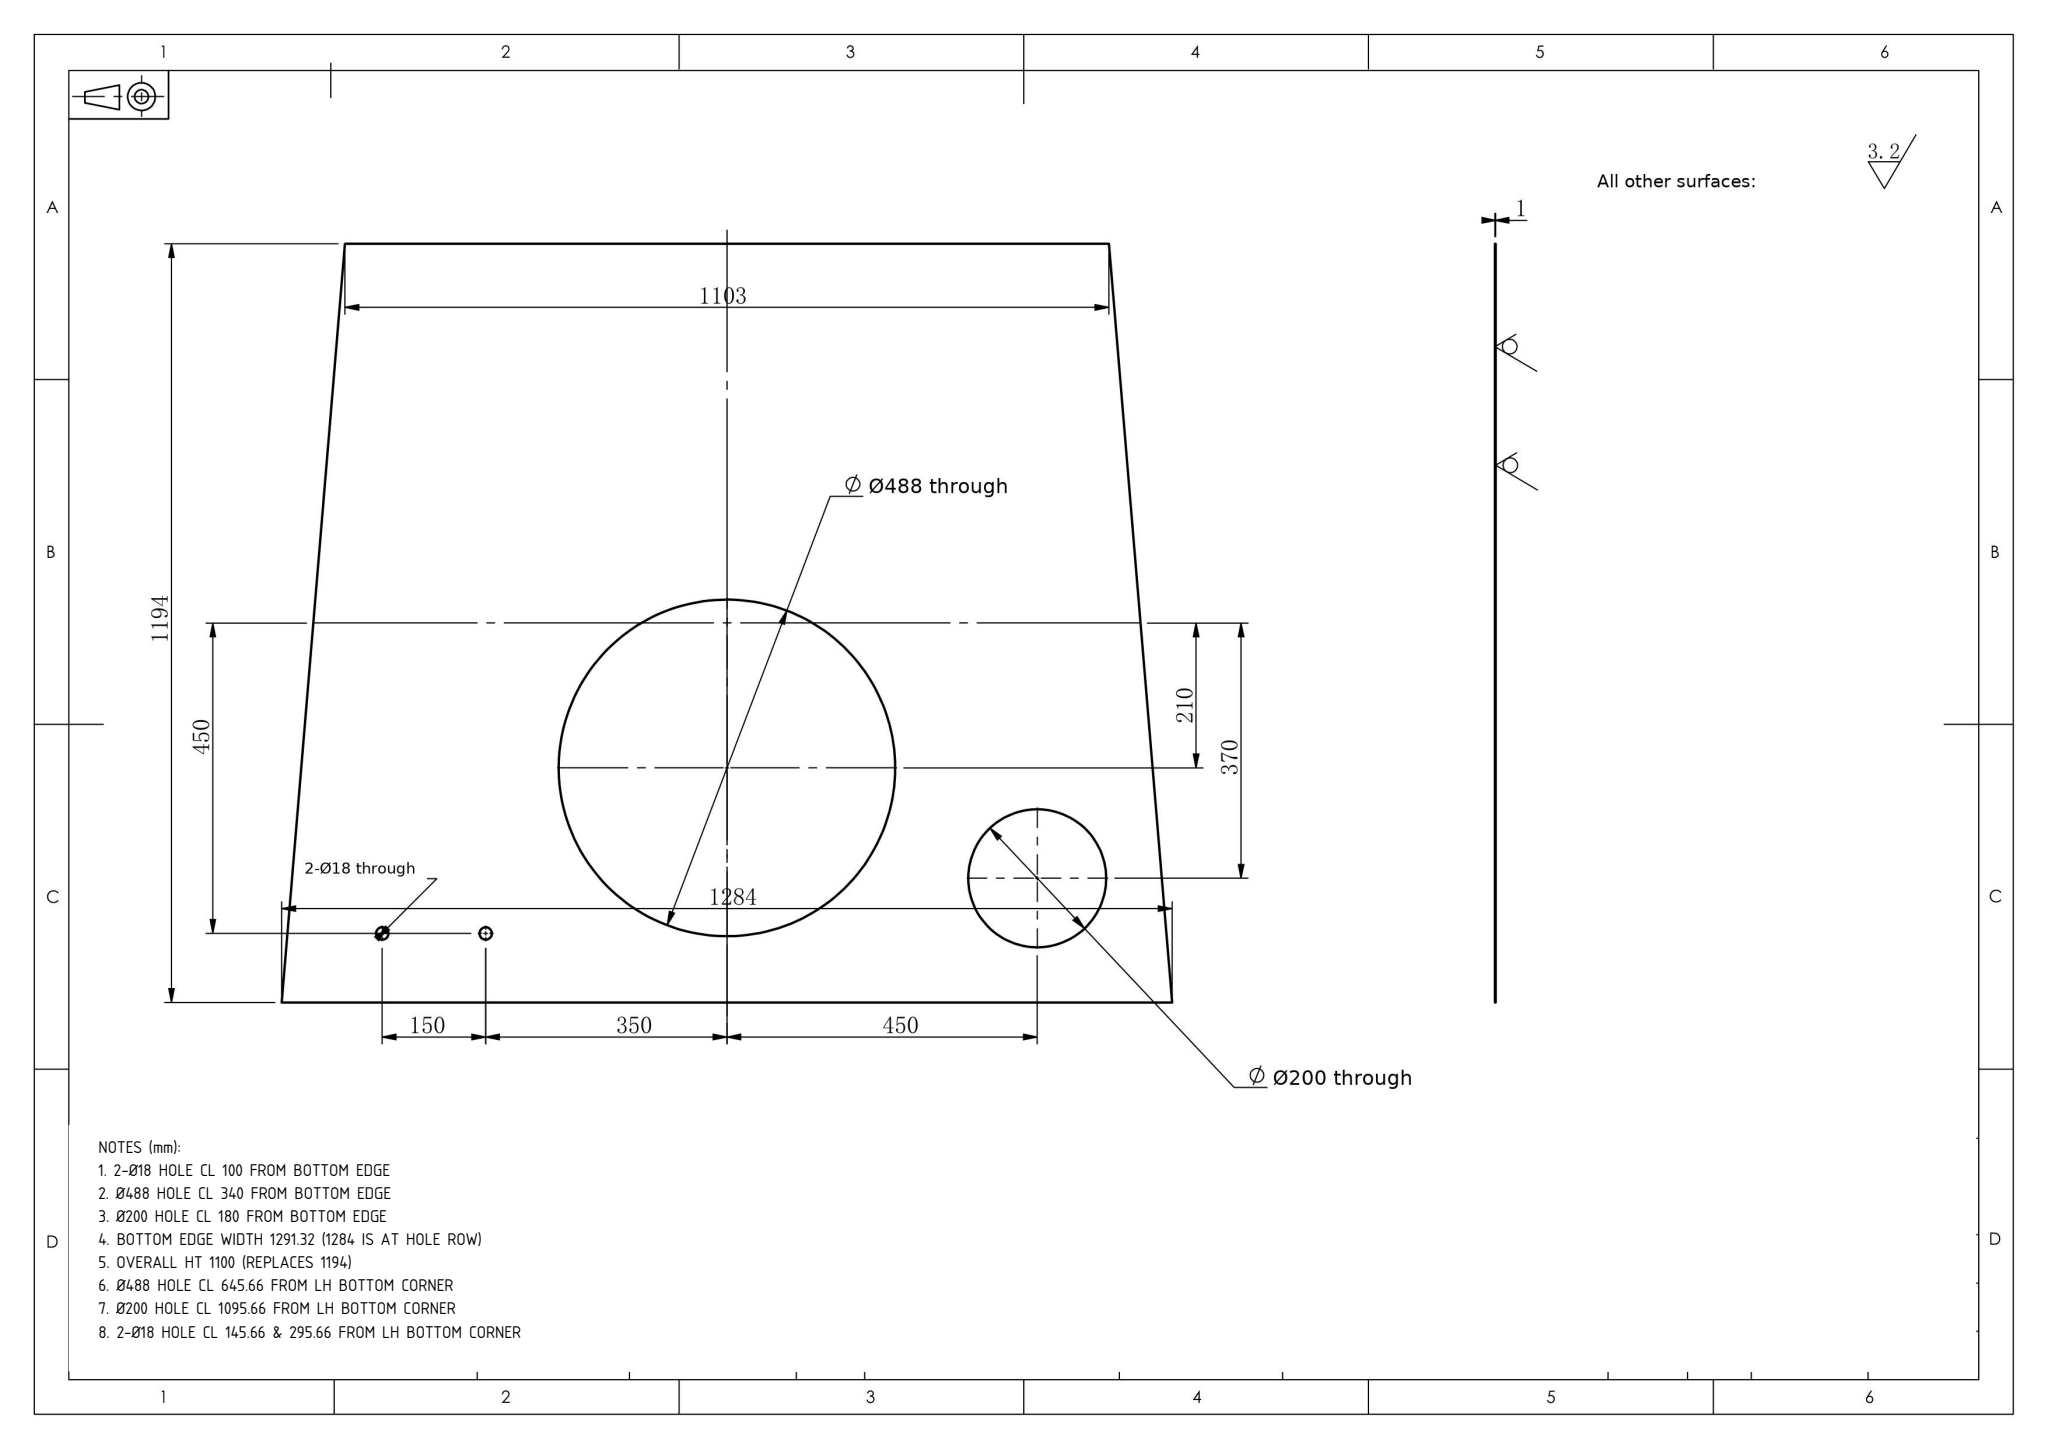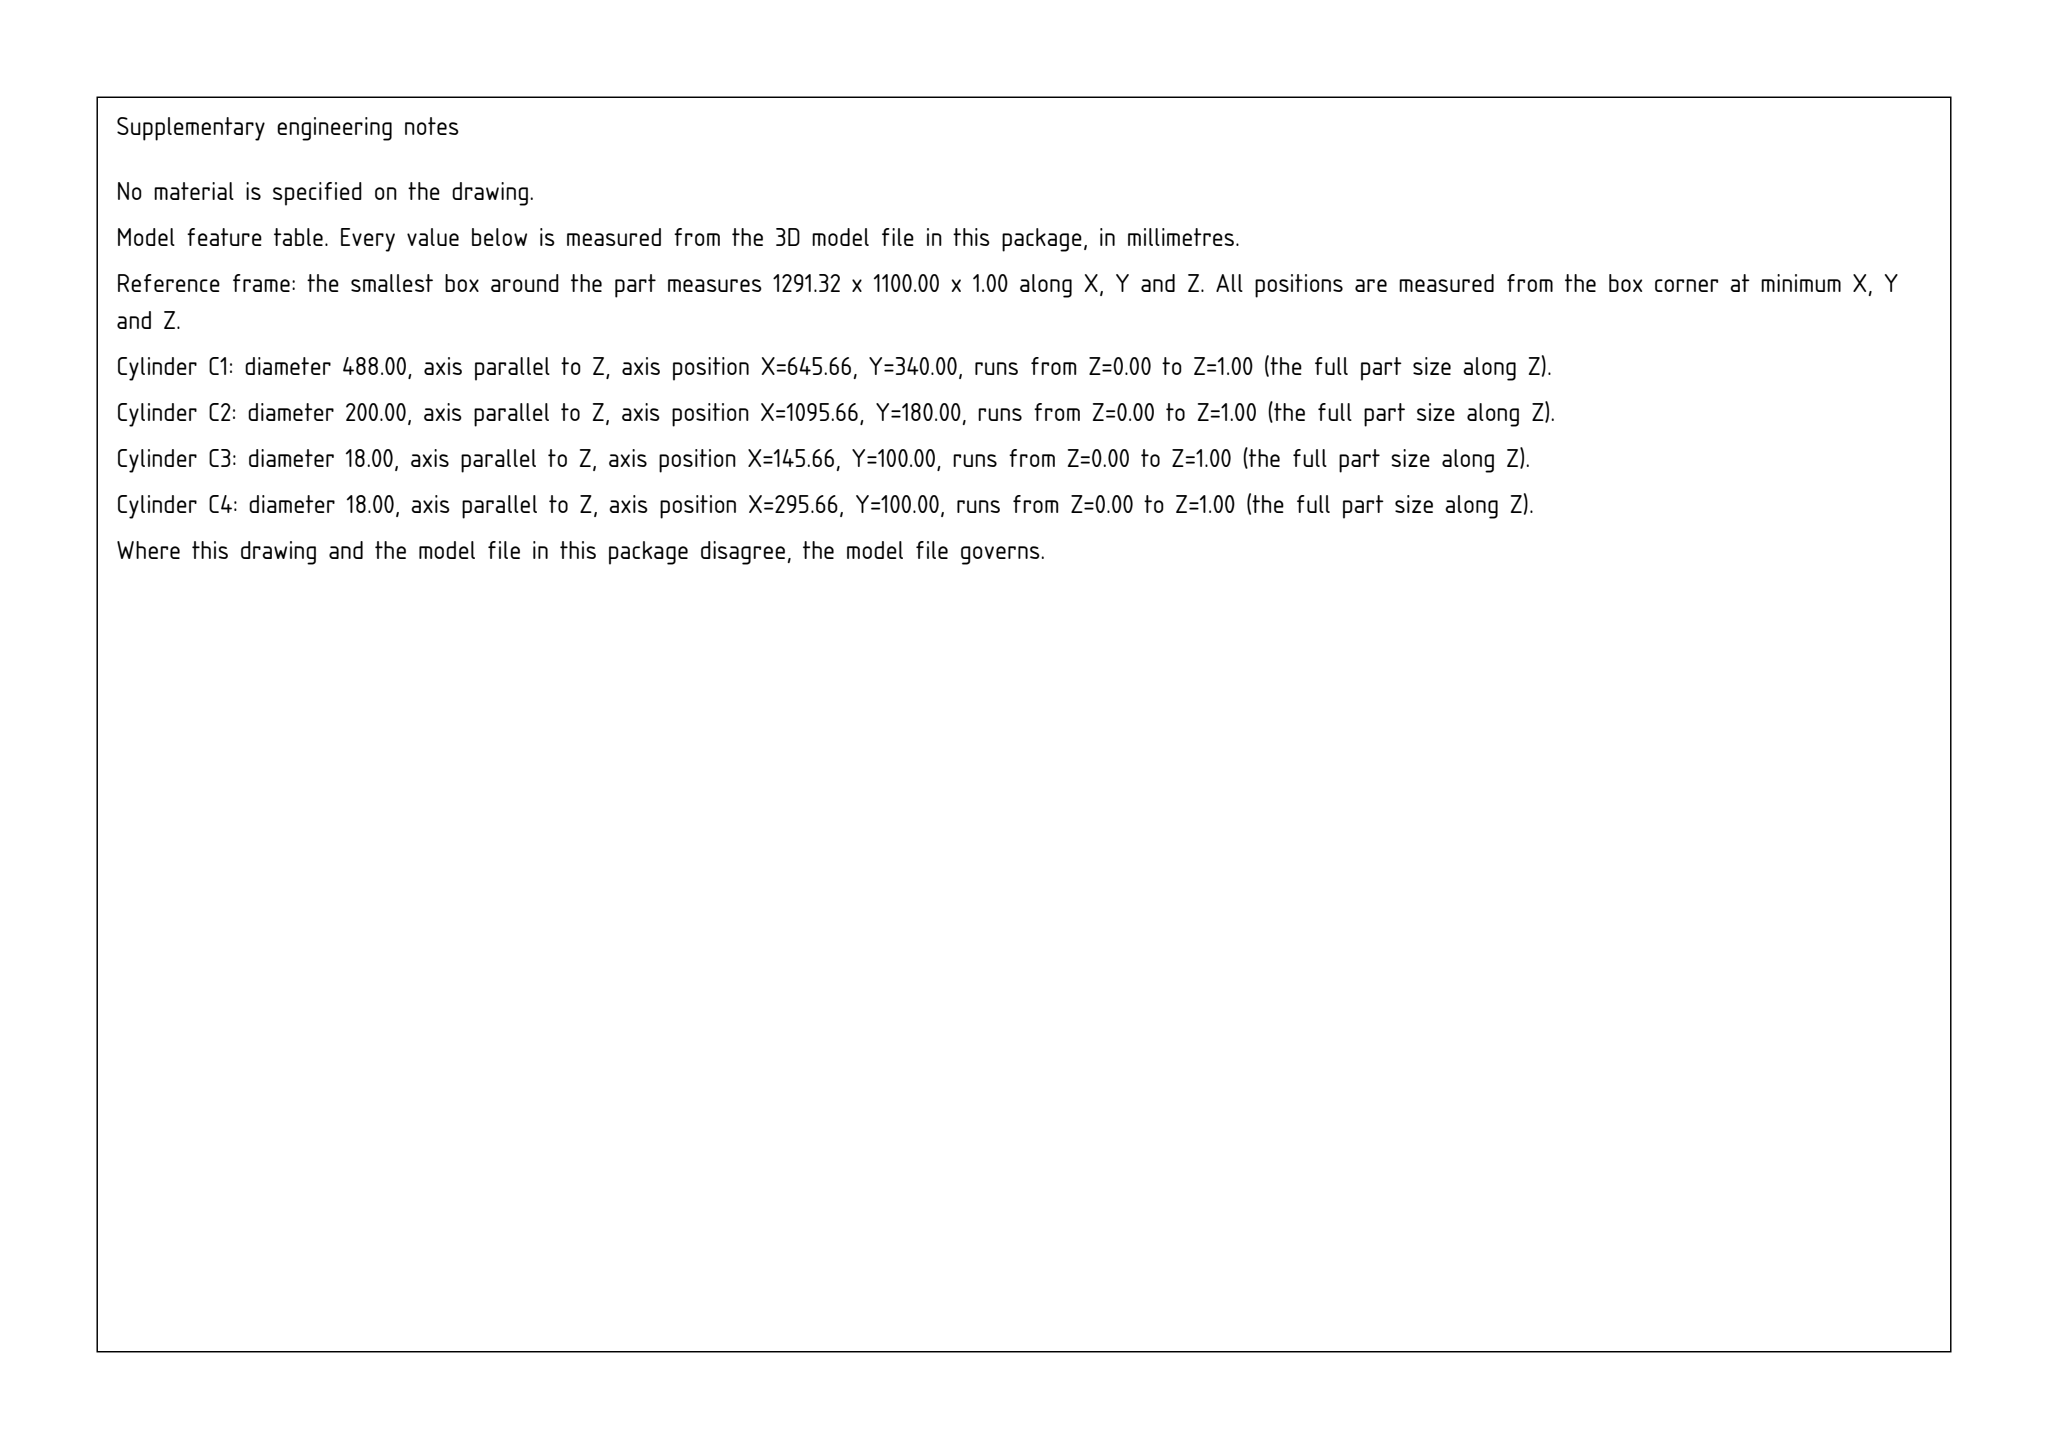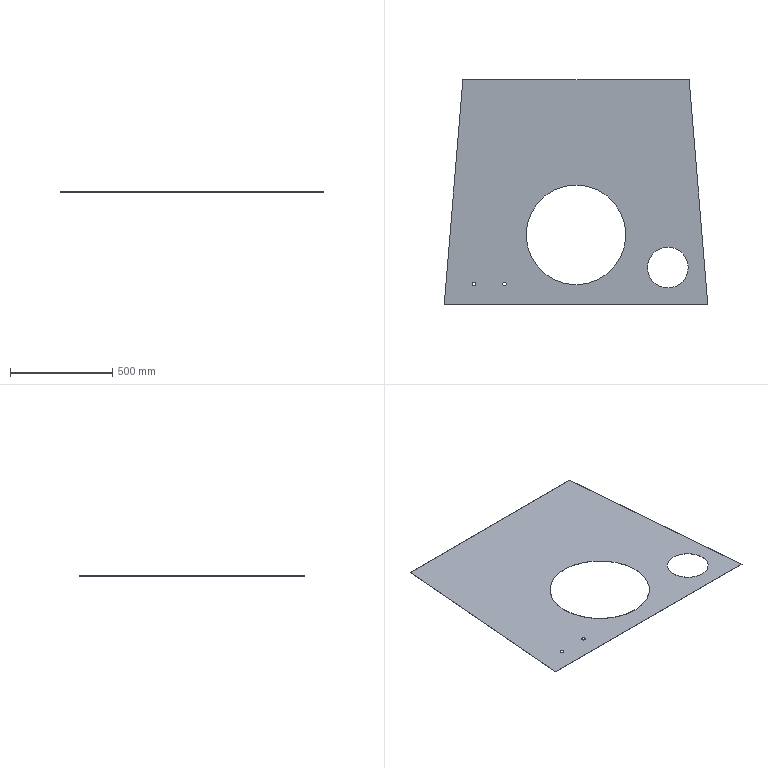Part | SolidWorks | mm | 1 solid | 14 faces | box 1291.32 x 1100 x 1 mm | volume 1100656 mm3 | cylinder 8 | plane 6 | commonest cylinder face diameters 18 x4 200 x2 488 x2
Drawing notes:
2-Ø18 HOLE CL 100 FROM BOTTOM EDGE | from the solid: Ø18 cyls at y=100.0, bbox y min=0 (bottom edge)
Ø488 HOLE CL 340 FROM BOTTOM EDGE | from the solid: Ø488 cyl pos y=340.0 from bbox min corner
Ø200 HOLE CL 180 FROM BOTTOM EDGE | from the solid: Ø200 cyl pos y=180.0 from bbox min corner
BOTTOM EDGE WIDTH 1291.32 (1284 IS AT HOLE ROW) | from the solid: bbox_xyz x=1291.32 at y=0 plane
OVERALL HT 1100 (REPLACES 1194) | from the solid: bbox_xyz y=1100.0; planes y=0 and y=1100
Ø488 HOLE CL 645.66 FROM LH BOTTOM CORNER | from the solid: Ø488 cyl pos x=645.66
Ø200 HOLE CL 1095.66 FROM LH BOTTOM CORNER | from the solid: Ø200 cyl pos x=1095.66
2-Ø18 HOLE CL 145.66 & 295.66 FROM LH BOTTOM CORNER | from the solid: Ø18 cyls x=145.66, 295.66
build123d program:
from build123d import *

# Parameters (mm, degrees)
SKETCH1_R           = 244
SKETCH1_R_2         = 100
SKETCH1_R_3         = 9
BOSS_EXTRUDE1_DEPTH = 1
SKETCH2_R           = 9
CUT_EXTRUDE1_DEPTH  = 10


with BuildPart() as part:
    # Sketch1 → Boss-Extrude1 (new body)
    with BuildSketch(Plane.XY):
        Polygon((1042.115, 1117.814), (-65.872, 1117.814), (-157.538, 17.814), (1133.782, 17.814), align=None)
        with Locations((488.122, 357.814)):
            Circle(SKETCH1_R, mode=Mode.SUBTRACT)
        with Locations((938.122, 197.814)):
            Circle(SKETCH1_R_2, mode=Mode.SUBTRACT)
        with Locations((-11.878, 117.814)):
            Circle(SKETCH1_R_3, mode=Mode.SUBTRACT)
    extrude(amount=BOSS_EXTRUDE1_DEPTH)

    # Sketch2 → Cut-Extrude1 (cut)
    with BuildSketch(Plane(origin=(0, 0, 0), x_dir=(-1, 0, 0), z_dir=(0, 0, -1))):
        with Locations((-138.122, 117.814)):
            Circle(SKETCH2_R)
    extrude(amount=-CUT_EXTRUDE1_DEPTH, mode=Mode.SUBTRACT)


solid = part.part
STEP:
#1=CARTESIAN_POINT('',(147.122,117.814,1.));
#2=VERTEX_POINT('',#1);
#3=CARTESIAN_POINT('',(129.122,117.814,1.));
#4=VERTEX_POINT('',#3);
#5=CARTESIAN_POINT('',(138.122,117.814,1.));
#6=DIRECTION('',(0.,0.,-1.));
#7=DIRECTION('',(-1.,0.,0.));
#8=AXIS2_PLACEMENT_3D('',#5,#6,#7);
#9=CIRCLE('',#8,9.);
#10=EDGE_CURVE('',#2,#4,#9,.T.);
#11=ORIENTED_EDGE('',*,*,#10,.F.);
#12=CARTESIAN_POINT('',(147.122,117.814,0.));
#13=VERTEX_POINT('',#12);
#14=CARTESIAN_POINT('',(147.122,117.814,10.));
#15=DIRECTION('',(0.,0.,-1.));
#16=VECTOR('',#15,1000.);
#17=LINE('',#14,#16);
#18=EDGE_CURVE('',#2,#13,#17,.T.);
#19=ORIENTED_EDGE('',*,*,#18,.T.);
#20=CARTESIAN_POINT('',(129.122,117.814,0.));
#21=VERTEX_POINT('',#20);
#22=CARTESIAN_POINT('',(138.122,117.814,0.));
#23=DIRECTION('',(0.,0.,-1.));
#24=DIRECTION('',(-1.,0.,0.));
#25=AXIS2_PLACEMENT_3D('',#22,#23,#24);
#26=CIRCLE('',#25,9.);
#27=EDGE_CURVE('',#13,#21,#26,.T.);
#28=ORIENTED_EDGE('',*,*,#27,.T.);
#29=CARTESIAN_POINT('',(129.122,117.814,10.));
#30=DIRECTION('',(0.,0.,-1.));
#31=VECTOR('',#30,1000.);
#32=LINE('',#29,#31);
#33=EDGE_CURVE('',#4,#21,#32,.T.);
#34=ORIENTED_EDGE('',*,*,#33,.F.);
#35=EDGE_LOOP('',(#11,#19,#28,#34));
#36=FACE_OUTER_BOUND('',#35,.T.);
#37=CARTESIAN_POINT('',(138.122,117.814,10.));
#38=DIRECTION('',(0.,0.,-1.));
#39=DIRECTION('',(-1.,0.,0.));
#40=AXIS2_PLACEMENT_3D('',#37,#38,#39);
#41=CYLINDRICAL_SURFACE('',#40,9.);
#42=ADVANCED_FACE('',(#36),#41,.F.);
#43=CARTESIAN_POINT('',(-20.878,117.814,1.));
#44=VERTEX_POINT('',#43);
#45=CARTESIAN_POINT('',(-2.878,117.814,1.));
#46=VERTEX_POINT('',#45);
#47=CARTESIAN_POINT('',(-11.878,117.814,1.));
#48=DIRECTION('',(0.,0.,1.));
#49=DIRECTION('',(1.,0.,0.));
#50=AXIS2_PLACEMENT_3D('',#47,#48,#49);
#51=CIRCLE('',#50,9.);
#52=EDGE_CURVE('',#44,#46,#51,.T.);
#53=ORIENTED_EDGE('',*,*,#52,.T.);
#54=CARTESIAN_POINT('',(-2.878,117.814,0.));
#55=VERTEX_POINT('',#54);
#56=CARTESIAN_POINT('',(-2.878,117.814,1.));
#57=DIRECTION('',(0.,0.,-1.));
#58=VECTOR('',#57,1000.);
#59=LINE('',#56,#58);
#60=EDGE_CURVE('',#46,#55,#59,.T.);
#61=ORIENTED_EDGE('',*,*,#60,.T.);
#62=CARTESIAN_POINT('',(-20.878,117.814,0.));
#63=VERTEX_POINT('',#62);
#64=CARTESIAN_POINT('',(-11.878,117.814,0.));
#65=DIRECTION('',(0.,0.,1.));
#66=DIRECTION('',(1.,0.,0.));
#67=AXIS2_PLACEMENT_3D('',#64,#65,#66);
#68=CIRCLE('',#67,9.);
#69=EDGE_CURVE('',#63,#55,#68,.T.);
#70=ORIENTED_EDGE('',*,*,#69,.F.);
#71=CARTESIAN_POINT('',(-20.878,117.814,1.));
#72=DIRECTION('',(0.,0.,-1.));
#73=VECTOR('',#72,1000.);
#74=LINE('',#71,#73);
#75=EDGE_CURVE('',#44,#63,#74,.T.);
#76=ORIENTED_EDGE('',*,*,#75,.F.);
#77=EDGE_LOOP('',(#53,#61,#70,#76));
#78=FACE_OUTER_BOUND('',#77,.T.);
#79=CARTESIAN_POINT('',(-11.878,117.814,1.));
#80=DIRECTION('',(0.,0.,-1.));
#81=DIRECTION('',(-1.,0.,0.));
#82=AXIS2_PLACEMENT_3D('',#79,#80,#81);
#83=CYLINDRICAL_SURFACE('',#82,9.);
#84=ADVANCED_FACE('',(#78),#83,.F.);
#85=CARTESIAN_POINT('',(838.122,197.814,1.));
#86=VERTEX_POINT('',#85);
#87=CARTESIAN_POINT('',(1038.122,197.814,1.));
#88=VERTEX_POINT('',#87);
#89=CARTESIAN_POINT('',(938.122,197.814,1.));
#90=DIRECTION('',(0.,0.,1.));
#91=DIRECTION('',(1.,0.,0.));
#92=AXIS2_PLACEMENT_3D('',#89,#90,#91);
#93=CIRCLE('',#92,100.);
#94=EDGE_CURVE('',#86,#88,#93,.T.);
#95=ORIENTED_EDGE('',*,*,#94,.T.);
#96=CARTESIAN_POINT('',(1038.122,197.814,0.));
#97=VERTEX_POINT('',#96);
#98=CARTESIAN_POINT('',(1038.122,197.814,1.));
#99=DIRECTION('',(0.,0.,-1.));
#100=VECTOR('',#99,1000.);
#101=LINE('',#98,#100);
#102=EDGE_CURVE('',#88,#97,#101,.T.);
#103=ORIENTED_EDGE('',*,*,#102,.T.);
#104=CARTESIAN_POINT('',(838.122,197.814,0.));
#105=VERTEX_POINT('',#104);
#106=CARTESIAN_POINT('',(938.122,197.814,0.));
#107=DIRECTION('',(0.,0.,1.));
#108=DIRECTION('',(1.,0.,0.));
#109=AXIS2_PLACEMENT_3D('',#106,#107,#108);
#110=CIRCLE('',#109,100.);
#111=EDGE_CURVE('',#105,#97,#110,.T.);
#112=ORIENTED_EDGE('',*,*,#111,.F.);
#113=CARTESIAN_POINT('',(838.122,197.814,1.));
#114=DIRECTION('',(0.,0.,-1.));
#115=VECTOR('',#114,1000.);
#116=LINE('',#113,#115);
#117=EDGE_CURVE('',#86,#105,#116,.T.);
#118=ORIENTED_EDGE('',*,*,#117,.F.);
#119=EDGE_LOOP('',(#95,#103,#112,#118));
#120=FACE_OUTER_BOUND('',#119,.T.);
#121=CARTESIAN_POINT('',(938.122,197.814,1.));
#122=DIRECTION('',(0.,0.,-1.));
#123=DIRECTION('',(-1.,0.,0.));
#124=AXIS2_PLACEMENT_3D('',#121,#122,#123);
#125=CYLINDRICAL_SURFACE('',#124,100.);
#126=ADVANCED_FACE('',(#120),#125,.F.);
#127=CARTESIAN_POINT('',(244.122,357.814,1.));
#128=VERTEX_POINT('',#127);
#129=CARTESIAN_POINT('',(732.122,357.814,1.));
#130=VERTEX_POINT('',#129);
#131=CARTESIAN_POINT('',(488.122,357.814,1.));
#132=DIRECTION('',(0.,0.,1.));
#133=DIRECTION('',(1.,0.,0.));
#134=AXIS2_PLACEMENT_3D('',#131,#132,#133);
#135=CIRCLE('',#134,244.);
#136=EDGE_CURVE('',#128,#130,#135,.T.);
#137=ORIENTED_EDGE('',*,*,#136,.T.);
#138=CARTESIAN_POINT('',(732.122,357.814,0.));
#139=VERTEX_POINT('',#138);
#140=CARTESIAN_POINT('',(732.122,357.814,1.));
#141=DIRECTION('',(0.,0.,-1.));
#142=VECTOR('',#141,1000.);
#143=LINE('',#140,#142);
#144=EDGE_CURVE('',#130,#139,#143,.T.);
#145=ORIENTED_EDGE('',*,*,#144,.T.);
#146=CARTESIAN_POINT('',(244.122,357.814,0.));
#147=VERTEX_POINT('',#146);
#148=CARTESIAN_POINT('',(488.122,357.814,0.));
#149=DIRECTION('',(0.,0.,1.));
#150=DIRECTION('',(1.,0.,0.));
#151=AXIS2_PLACEMENT_3D('',#148,#149,#150);
#152=CIRCLE('',#151,244.);
#153=EDGE_CURVE('',#147,#139,#152,.T.);
#154=ORIENTED_EDGE('',*,*,#153,.F.);
#155=CARTESIAN_POINT('',(244.122,357.814,1.));
#156=DIRECTION('',(0.,0.,-1.));
#157=VECTOR('',#156,1000.);
#158=LINE('',#155,#157);
#159=EDGE_CURVE('',#128,#147,#158,.T.);
#160=ORIENTED_EDGE('',*,*,#159,.F.);
#161=EDGE_LOOP('',(#137,#145,#154,#160));
#162=FACE_OUTER_BOUND('',#161,.T.);
#163=CARTESIAN_POINT('',(488.122,357.814,1.));
#164=DIRECTION('',(0.,0.,-1.));
#165=DIRECTION('',(-1.,0.,0.));
#166=AXIS2_PLACEMENT_3D('',#163,#164,#165);
#167=CYLINDRICAL_SURFACE('',#166,244.);
#168=ADVANCED_FACE('',(#162),#167,.F.);
#169=CARTESIAN_POINT('',(138.122,117.814,1.));
#170=DIRECTION('',(0.,0.,-1.));
#171=DIRECTION('',(-1.,0.,0.));
#172=AXIS2_PLACEMENT_3D('',#169,#170,#171);
#173=CIRCLE('',#172,9.);
#174=EDGE_CURVE('',#4,#2,#173,.T.);
#175=ORIENTED_EDGE('',*,*,#174,.T.);
#176=ORIENTED_EDGE('',*,*,#10,.T.);
#177=EDGE_LOOP('',(#175,#176));
#178=FACE_BOUND('',#177,.T.);
#179=CARTESIAN_POINT('',(1133.782,17.814,1.));
#180=VERTEX_POINT('',#179);
#181=CARTESIAN_POINT('',(1042.115,1117.814,1.));
#182=VERTEX_POINT('',#181);
#183=CARTESIAN_POINT('',(1042.115,1117.814,1.));
#184=DIRECTION('',(-0.08305,0.9965,0.));
#185=VECTOR('',#184,1000.);
#186=LINE('',#183,#185);
#187=EDGE_CURVE('',#180,#182,#186,.T.);
#188=ORIENTED_EDGE('',*,*,#187,.T.);
#189=CARTESIAN_POINT('',(-65.872,1117.814,1.));
#190=VERTEX_POINT('',#189);
#191=CARTESIAN_POINT('',(1042.115,1117.814,1.));
#192=DIRECTION('',(-1.,-0.,0.));
#193=VECTOR('',#192,1000.);
#194=LINE('',#191,#193);
#195=EDGE_CURVE('',#182,#190,#194,.T.);
#196=ORIENTED_EDGE('',*,*,#195,.T.);
#197=CARTESIAN_POINT('',(-157.538,17.814,1.));
#198=VERTEX_POINT('',#197);
#199=CARTESIAN_POINT('',(-65.872,1117.814,1.));
#200=DIRECTION('',(-0.08305,-0.9965,0.));
#201=VECTOR('',#200,1000.);
#202=LINE('',#199,#201);
#203=EDGE_CURVE('',#190,#198,#202,.T.);
#204=ORIENTED_EDGE('',*,*,#203,.T.);
#205=CARTESIAN_POINT('',(1133.782,17.814,1.));
#206=DIRECTION('',(1.,0.,0.));
#207=VECTOR('',#206,1000.);
#208=LINE('',#205,#207);
#209=EDGE_CURVE('',#198,#180,#208,.T.);
#210=ORIENTED_EDGE('',*,*,#209,.T.);
#211=EDGE_LOOP('',(#188,#196,#204,#210));
#212=FACE_OUTER_BOUND('',#211,.T.);
#213=ORIENTED_EDGE('',*,*,#136,.F.);
#214=CARTESIAN_POINT('',(488.122,357.814,1.));
#215=DIRECTION('',(0.,0.,1.));
#216=DIRECTION('',(1.,0.,0.));
#217=AXIS2_PLACEMENT_3D('',#214,#215,#216);
#218=CIRCLE('',#217,244.);
#219=EDGE_CURVE('',#130,#128,#218,.T.);
#220=ORIENTED_EDGE('',*,*,#219,.F.);
#221=EDGE_LOOP('',(#213,#220));
#222=FACE_BOUND('',#221,.T.);
#223=ORIENTED_EDGE('',*,*,#94,.F.);
#224=CARTESIAN_POINT('',(938.122,197.814,1.));
#225=DIRECTION('',(0.,0.,1.));
#226=DIRECTION('',(1.,0.,0.));
#227=AXIS2_PLACEMENT_3D('',#224,#225,#226);
#228=CIRCLE('',#227,100.);
#229=EDGE_CURVE('',#88,#86,#228,.T.);
#230=ORIENTED_EDGE('',*,*,#229,.F.);
#231=EDGE_LOOP('',(#223,#230));
#232=FACE_BOUND('',#231,.T.);
#233=ORIENTED_EDGE('',*,*,#52,.F.);
#234=CARTESIAN_POINT('',(-11.878,117.814,1.));
#235=DIRECTION('',(0.,0.,1.));
#236=DIRECTION('',(1.,0.,0.));
#237=AXIS2_PLACEMENT_3D('',#234,#235,#236);
#238=CIRCLE('',#237,9.);
#239=EDGE_CURVE('',#46,#44,#238,.T.);
#240=ORIENTED_EDGE('',*,*,#239,.F.);
#241=EDGE_LOOP('',(#233,#240));
#242=FACE_BOUND('',#241,.T.);
#243=CARTESIAN_POINT('',(1133.782,17.814,1.));
#244=DIRECTION('',(0.,0.,-1.));
#245=DIRECTION('',(-1.,0.,0.));
#246=AXIS2_PLACEMENT_3D('',#243,#244,#245);
#247=PLANE('',#246);
#248=ADVANCED_FACE('',(#178,#212,#222,#232,#242),#247,.F.);
#249=CARTESIAN_POINT('',(138.122,117.814,0.));
#250=DIRECTION('',(0.,0.,-1.));
#251=DIRECTION('',(-1.,0.,0.));
#252=AXIS2_PLACEMENT_3D('',#249,#250,#251);
#253=CIRCLE('',#252,9.);
#254=EDGE_CURVE('',#21,#13,#253,.T.);
#255=ORIENTED_EDGE('',*,*,#254,.F.);
#256=ORIENTED_EDGE('',*,*,#27,.F.);
#257=EDGE_LOOP('',(#255,#256));
#258=FACE_BOUND('',#257,.T.);
#259=ORIENTED_EDGE('',*,*,#111,.T.);
#260=CARTESIAN_POINT('',(938.122,197.814,0.));
#261=DIRECTION('',(0.,0.,1.));
#262=DIRECTION('',(1.,0.,0.));
#263=AXIS2_PLACEMENT_3D('',#260,#261,#262);
#264=CIRCLE('',#263,100.);
#265=EDGE_CURVE('',#97,#105,#264,.T.);
#266=ORIENTED_EDGE('',*,*,#265,.T.);
#267=EDGE_LOOP('',(#259,#266));
#268=FACE_BOUND('',#267,.T.);
#269=CARTESIAN_POINT('',(1133.782,17.814,0.));
#270=VERTEX_POINT('',#269);
#271=CARTESIAN_POINT('',(1042.115,1117.814,0.));
#272=VERTEX_POINT('',#271);
#273=CARTESIAN_POINT('',(1042.115,1117.814,0.));
#274=DIRECTION('',(-0.08305,0.9965,0.));
#275=VECTOR('',#274,1000.);
#276=LINE('',#273,#275);
#277=EDGE_CURVE('',#270,#272,#276,.T.);
#278=ORIENTED_EDGE('',*,*,#277,.F.);
#279=CARTESIAN_POINT('',(-157.538,17.814,0.));
#280=VERTEX_POINT('',#279);
#281=CARTESIAN_POINT('',(1133.782,17.814,0.));
#282=DIRECTION('',(1.,0.,0.));
#283=VECTOR('',#282,1000.);
#284=LINE('',#281,#283);
#285=EDGE_CURVE('',#280,#270,#284,.T.);
#286=ORIENTED_EDGE('',*,*,#285,.F.);
#287=CARTESIAN_POINT('',(-65.872,1117.814,0.));
#288=VERTEX_POINT('',#287);
#289=CARTESIAN_POINT('',(-65.872,1117.814,0.));
#290=DIRECTION('',(-0.08305,-0.9965,0.));
#291=VECTOR('',#290,1000.);
#292=LINE('',#289,#291);
#293=EDGE_CURVE('',#288,#280,#292,.T.);
#294=ORIENTED_EDGE('',*,*,#293,.F.);
#295=CARTESIAN_POINT('',(1042.115,1117.814,0.));
#296=DIRECTION('',(-1.,-0.,0.));
#297=VECTOR('',#296,1000.);
#298=LINE('',#295,#297);
#299=EDGE_CURVE('',#272,#288,#298,.T.);
#300=ORIENTED_EDGE('',*,*,#299,.F.);
#301=EDGE_LOOP('',(#278,#286,#294,#300));
#302=FACE_OUTER_BOUND('',#301,.T.);
#303=ORIENTED_EDGE('',*,*,#153,.T.);
#304=CARTESIAN_POINT('',(488.122,357.814,0.));
#305=DIRECTION('',(0.,0.,1.));
#306=DIRECTION('',(1.,0.,0.));
#307=AXIS2_PLACEMENT_3D('',#304,#305,#306);
#308=CIRCLE('',#307,244.);
#309=EDGE_CURVE('',#139,#147,#308,.T.);
#310=ORIENTED_EDGE('',*,*,#309,.T.);
#311=EDGE_LOOP('',(#303,#310));
#312=FACE_BOUND('',#311,.T.);
#313=ORIENTED_EDGE('',*,*,#69,.T.);
#314=CARTESIAN_POINT('',(-11.878,117.814,0.));
#315=DIRECTION('',(0.,0.,1.));
#316=DIRECTION('',(1.,0.,0.));
#317=AXIS2_PLACEMENT_3D('',#314,#315,#316);
#318=CIRCLE('',#317,9.);
#319=EDGE_CURVE('',#55,#63,#318,.T.);
#320=ORIENTED_EDGE('',*,*,#319,.T.);
#321=EDGE_LOOP('',(#313,#320));
#322=FACE_BOUND('',#321,.T.);
#323=CARTESIAN_POINT('',(1133.782,17.814,0.));
#324=DIRECTION('',(0.,0.,-1.));
#325=DIRECTION('',(-1.,0.,0.));
#326=AXIS2_PLACEMENT_3D('',#323,#324,#325);
#327=PLANE('',#326);
#328=ADVANCED_FACE('',(#258,#268,#302,#312,#322),#327,.T.);
#329=ORIENTED_EDGE('',*,*,#277,.T.);
#330=CARTESIAN_POINT('',(1042.115,1117.814,1.));
#331=DIRECTION('',(0.,0.,-1.));
#332=VECTOR('',#331,1000.);
#333=LINE('',#330,#332);
#334=EDGE_CURVE('',#182,#272,#333,.T.);
#335=ORIENTED_EDGE('',*,*,#334,.F.);
#336=ORIENTED_EDGE('',*,*,#187,.F.);
#337=CARTESIAN_POINT('',(1133.782,17.814,1.));
#338=DIRECTION('',(0.,0.,-1.));
#339=VECTOR('',#338,1000.);
#340=LINE('',#337,#339);
#341=EDGE_CURVE('',#180,#270,#340,.T.);
#342=ORIENTED_EDGE('',*,*,#341,.T.);
#343=EDGE_LOOP('',(#329,#335,#336,#342));
#344=FACE_OUTER_BOUND('',#343,.T.);
#345=CARTESIAN_POINT('',(1042.115,1117.814,1.));
#346=DIRECTION('',(-0.9965,-0.08305,0.));
#347=DIRECTION('',(0.08305,-0.9965,0.));
#348=AXIS2_PLACEMENT_3D('',#345,#346,#347);
#349=PLANE('',#348);
#350=ADVANCED_FACE('',(#344),#349,.F.);
#351=ORIENTED_EDGE('',*,*,#299,.T.);
#352=CARTESIAN_POINT('',(-65.872,1117.814,1.));
#353=DIRECTION('',(0.,0.,-1.));
#354=VECTOR('',#353,1000.);
#355=LINE('',#352,#354);
#356=EDGE_CURVE('',#190,#288,#355,.T.);
#357=ORIENTED_EDGE('',*,*,#356,.F.);
#358=ORIENTED_EDGE('',*,*,#195,.F.);
#359=ORIENTED_EDGE('',*,*,#334,.T.);
#360=EDGE_LOOP('',(#351,#357,#358,#359));
#361=FACE_OUTER_BOUND('',#360,.T.);
#362=CARTESIAN_POINT('',(1042.115,1117.814,1.));
#363=DIRECTION('',(0.,-1.,0.));
#364=DIRECTION('',(1.,0.,0.));
#365=AXIS2_PLACEMENT_3D('',#362,#363,#364);
#366=PLANE('',#365);
#367=ADVANCED_FACE('',(#361),#366,.F.);
#368=ORIENTED_EDGE('',*,*,#293,.T.);
#369=CARTESIAN_POINT('',(-157.538,17.814,1.));
#370=DIRECTION('',(0.,0.,-1.));
#371=VECTOR('',#370,1000.);
#372=LINE('',#369,#371);
#373=EDGE_CURVE('',#198,#280,#372,.T.);
#374=ORIENTED_EDGE('',*,*,#373,.F.);
#375=ORIENTED_EDGE('',*,*,#203,.F.);
#376=ORIENTED_EDGE('',*,*,#356,.T.);
#377=EDGE_LOOP('',(#368,#374,#375,#376));
#378=FACE_OUTER_BOUND('',#377,.T.);
#379=CARTESIAN_POINT('',(-65.872,1117.814,1.));
#380=DIRECTION('',(0.9965,-0.08305,0.));
#381=DIRECTION('',(0.08305,0.9965,0.));
#382=AXIS2_PLACEMENT_3D('',#379,#380,#381);
#383=PLANE('',#382);
#384=ADVANCED_FACE('',(#378),#383,.F.);
#385=ORIENTED_EDGE('',*,*,#285,.T.);
#386=ORIENTED_EDGE('',*,*,#341,.F.);
#387=ORIENTED_EDGE('',*,*,#209,.F.);
#388=ORIENTED_EDGE('',*,*,#373,.T.);
#389=EDGE_LOOP('',(#385,#386,#387,#388));
#390=FACE_OUTER_BOUND('',#389,.T.);
#391=CARTESIAN_POINT('',(1133.782,17.814,1.));
#392=DIRECTION('',(-0.,1.,0.));
#393=DIRECTION('',(-1.,-0.,0.));
#394=AXIS2_PLACEMENT_3D('',#391,#392,#393);
#395=PLANE('',#394);
#396=ADVANCED_FACE('',(#390),#395,.F.);
#397=ORIENTED_EDGE('',*,*,#144,.F.);
#398=ORIENTED_EDGE('',*,*,#219,.T.);
#399=ORIENTED_EDGE('',*,*,#159,.T.);
#400=ORIENTED_EDGE('',*,*,#309,.F.);
#401=EDGE_LOOP('',(#397,#398,#399,#400));
#402=FACE_OUTER_BOUND('',#401,.T.);
#403=CARTESIAN_POINT('',(488.122,357.814,1.));
#404=DIRECTION('',(0.,0.,-1.));
#405=DIRECTION('',(-1.,0.,0.));
#406=AXIS2_PLACEMENT_3D('',#403,#404,#405);
#407=CYLINDRICAL_SURFACE('',#406,244.);
#408=ADVANCED_FACE('',(#402),#407,.F.);
#409=ORIENTED_EDGE('',*,*,#102,.F.);
#410=ORIENTED_EDGE('',*,*,#229,.T.);
#411=ORIENTED_EDGE('',*,*,#117,.T.);
#412=ORIENTED_EDGE('',*,*,#265,.F.);
#413=EDGE_LOOP('',(#409,#410,#411,#412));
#414=FACE_OUTER_BOUND('',#413,.T.);
#415=CARTESIAN_POINT('',(938.122,197.814,1.));
#416=DIRECTION('',(0.,0.,-1.));
#417=DIRECTION('',(-1.,0.,0.));
#418=AXIS2_PLACEMENT_3D('',#415,#416,#417);
#419=CYLINDRICAL_SURFACE('',#418,100.);
#420=ADVANCED_FACE('',(#414),#419,.F.);
#421=ORIENTED_EDGE('',*,*,#60,.F.);
#422=ORIENTED_EDGE('',*,*,#239,.T.);
#423=ORIENTED_EDGE('',*,*,#75,.T.);
#424=ORIENTED_EDGE('',*,*,#319,.F.);
#425=EDGE_LOOP('',(#421,#422,#423,#424));
#426=FACE_OUTER_BOUND('',#425,.T.);
#427=CARTESIAN_POINT('',(-11.878,117.814,1.));
#428=DIRECTION('',(0.,0.,-1.));
#429=DIRECTION('',(-1.,0.,0.));
#430=AXIS2_PLACEMENT_3D('',#427,#428,#429);
#431=CYLINDRICAL_SURFACE('',#430,9.);
#432=ADVANCED_FACE('',(#426),#431,.F.);
#433=ORIENTED_EDGE('',*,*,#18,.F.);
#434=ORIENTED_EDGE('',*,*,#174,.F.);
#435=ORIENTED_EDGE('',*,*,#33,.T.);
#436=ORIENTED_EDGE('',*,*,#254,.T.);
#437=EDGE_LOOP('',(#433,#434,#435,#436));
#438=FACE_OUTER_BOUND('',#437,.T.);
#439=CARTESIAN_POINT('',(138.122,117.814,10.));
#440=DIRECTION('',(0.,0.,-1.));
#441=DIRECTION('',(-1.,0.,0.));
#442=AXIS2_PLACEMENT_3D('',#439,#440,#441);
#443=CYLINDRICAL_SURFACE('',#442,9.);
#444=ADVANCED_FACE('',(#438),#443,.F.);
#445=CLOSED_SHELL('',(#42,#84,#126,#168,#248,#328,#350,#367,#384,#396,#408,#420,#432,#444));
#446=MANIFOLD_SOLID_BREP('',#445);
#447=CARTESIAN_POINT('',(0.,0.,0.));
#448=DIRECTION('',(0.,0.,1.));
#449=DIRECTION('',(1.,0.,0.));
#450=AXIS2_PLACEMENT_3D('',#447,#448,#449);
#451=(LENGTH_UNIT()NAMED_UNIT(*)SI_UNIT(.MILLI.,.METRE.));
#452=UNCERTAINTY_MEASURE_WITH_UNIT(LENGTH_MEASURE(0.00001),#451,'','');
#453=(NAMED_UNIT(*)PLANE_ANGLE_UNIT()SI_UNIT($,.RADIAN.));
#454=(NAMED_UNIT(*)SI_UNIT($,.STERADIAN.)SOLID_ANGLE_UNIT());
#455=(GEOMETRIC_REPRESENTATION_CONTEXT(3)GLOBAL_UNCERTAINTY_ASSIGNED_CONTEXT((#452))GLOBAL_UNIT_ASSIGNED_CONTEXT((#451,#453,#454))REPRESENTATION_CONTEXT('',''));
#456=ADVANCED_BREP_SHAPE_REPRESENTATION('',(#446,#450),#455);